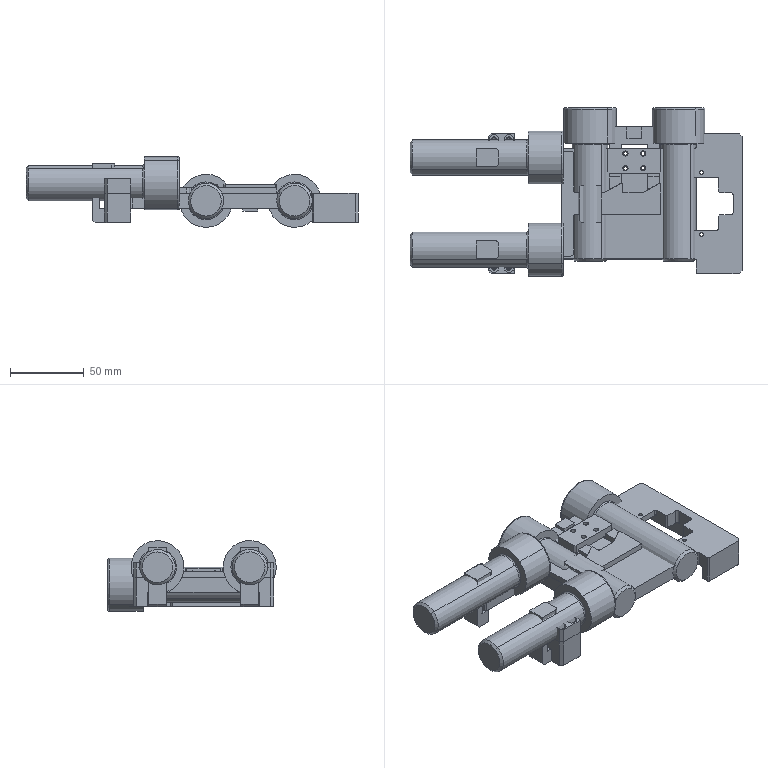Assembly | SolidWorks | mm | 19 component files | 19 solids | 652 faces | box 225 x 114.25 x 48 mm | volume 368375 mm3 | plane 378 | cylinder 216 | cone 34 | torus 16 | spline 8 | commonest cylinder face diameters 5.2 x36 2 x33 2.5 x28 8 x20 4.5 x16 4 x16 3.5 x12 3.3 x8
Bill of materials:
Baffle | 2 |  | Flat annular disc: a thin ring with a concentric through-bore, resembling a plain flat washer.
ClampB | 1 |  | Rectangular block with a stepped top. Two counterbored vertical through-holes sit on the top face, a large horizontal through-bore runs through one side face, and two corners are chamfered in plan.
ClampC | 1 |  | Flat rectangular plate with four through-holes in a rectangular pattern and four chamfered corners.
ConnectingRod | 1 |  | Thin flat profiled plate. A central bar ends in a C-shaped frame on one side, and the other end is a stepped tab with angled shoulders. Small upright posts stand at the four corners of the C-shape.
Jig | 1 |  | Large flat base plate, roughly H/U-shaped in plan, with thicker raised pads at the ends. It has many small and medium through-holes, a stepped rectangular cutout, and narrow slots or rails on the top face.
MirrorClampB1 | 1 |  | Rectangular block with a raised step running along the top. The lower step has two counterbored vertical through-holes, a large horizontal through-bore passes through the taller portion, and two corners are chamfered in plan.
MovingBlock | 2 |  | Bracket-like body: an upright with a rounded top cap, and a horizontal arm projecting sideways that ends in a short upturned tab with a small hole. A small block sits at the base.
PressurePlateA | 1 |  | Rectangular block with two counterbored-looking vertical holes and a wide rectangular channel cut through the underside, giving a bridge or inverted-U cross-section. All plan corners are chamfered.
SideMovingBlock | 1 |  | Complex machined bracket with a long main bar and two parallel legs (a Pi/comb shape in plan). It has multiple through-holes, including a larger central bore, plus end blocks with stepped faces and small raised pads.
socket head cap screw_iso | 4 |  | Cylindrical headed fastener-like part: a plain cylindrical shank with a chamfered tip and a larger cylindrical head with a hexagonal socket recess. It resembles a socket-head cap screw.
VUM5-30 | 2 |  | Open helical coil of round-section wire, about four turns at constant diameter and roughly uniform pitch, with plain cut ends; shape matches a helical coil spring.
VUM5-30 | 2 |  | Open helical coil of round-section wire, about four turns at constant diameter and uniform pitch, with plain flat cut ends; shape matches a helical coil spring, with wire that looks slightly thinner relative to the coil diameter than part-0.
Mates:
1. coincident | Jig-1 face at (-86, 27, 7) dir (0, 0, 1) | MovingBlock-1 face at (-64, 35.5, 7) dir (0, 0, -1)
2. coincident | Jig-1 face at (-86, 27, 7) dir (0, 1, 0) | MovingBlock-1 face at (-64, 27, 10) dir (0, -1, 0)
3. distance | MovingBlock-1 face at (-64, 35.5, 7) dir (1, 0, 0) | Jig-1 face at (-56, 35.5, 7) dir (-1, 0, 0)
4. coincident | Jig-1 face at (-86, 47.5, 10) dir (0, 0, 1) | ClampB-1 face at (-86, 25, 10) dir (0, 0, -1)
5. coincident | Jig-1 face at (-86, 25, 10) dir (0, -1, 0) | ClampB-1 face at (-86, 25, 20) dir (0, -1, 0)
6. coincident | Jig-1 face at (-86, -47.5, 10) dir (-1, 0, 0) | ClampB-1 face at (-86, 47.5, 10) dir (-1, 0, 0)
7. coincident | Jig-1 face at (-86, -27, 7) dir (0, 0, 1) | MovingBlock-2 face at (-64, -27, 7) dir (0, 0, -1)
8. coincident | Jig-1 face at (-86, -35.5, 7) dir (0, 1, 0) | MovingBlock-2 face at (-64, -35.5, 10) dir (0, -1, 0)
9. coincident | Jig-1 face at (-86, 47.5, 10) dir (0, 0, 1) | ConnectingRod-1 face at (-64, 35.5, 10) dir (0, 0, -1)
10. coincident | Jig-1 face at (22, 2.5, 5) dir (0, 0, 1) | SideMovingBlock-1 face at (-22, 40.098, 5) dir (0, 0, -1)
11. coincident | Jig-1 face at (-4, 37.5, 5) dir (1, 0, 0) | SideMovingBlock-1 face at (-4, 10.098, 5) dir (-1, 0, 0)
12. coincident | PressurePlateA-1 face at (-24, 12.5, 10) dir (0, 0, -1) | Jig-1 face at (-86, 47.5, 10) dir (0, 0, 1)
13. distance | PressurePlateA-1 face at (-24, -12.5, 10) dir (-1, 0, 0) | Jig-1 face at (-36, 25, 10) dir (-1, 0, 0)
14. distance | socket head cap screw_iso-4 face at (-17, 65, 5) dir (0, 1, 0) | Jig-1 face at (55, 37.5, 10) dir (0, 1, 0)
15. coincident | Jig-1 face at (-86, 47.5, 10) dir (0, 0, 1) | ClampC-1 face at (-5, 37.5, 10) dir (0, 0, -1)
16. coincident | Jig-1 face at (55, 37.5, 10) dir (0, 1, 0) | ClampC-1 face at (31, 37.5, 16) dir (0, 1, 0)
17. concentric | socket head cap screw_iso-3 face at (-3.25, 31.25, 17) dir (1, 0, 0) r 12 | MovingBlock-1 face at (-64, 31.25, 17) dir (1, 0, 0) r 1.25
18. coincident | MovingBlock-1 face at (-67, 27, 20) dir (-1, 0, 0) | VUM5-30-1 face at (-67, 23.7, 17.885) dir (1, 0, 0)
19. coincident | MovingBlock-1 face at (-94, 25.25, -10) dir (-1, 0, 0) | MovingBlock-2 face at (-94, -37.25, -10) dir (-1, 0, 0)
20. distance | socket head cap screw_iso-3 face at (-59, 44.866, 28.773) dir (-1, 0, 0) | MovingBlock-1 face at (-64, 35.5, 7) dir (1, 0, 0)
21. coincident | MovingBlock-1 face at (-64, 35.5, 7) dir (1, 0, 0) | ConnectingRod-1 face at (-64, -35.5, 14) dir (-1, 0, 0)
22. coincident | MovingBlock-1 face at (-64, 35.5, 10) dir (0, 1, 0) | ConnectingRod-1 face at (31, 35.5, 14) dir (0, 1, 0)
23. concentric | ClampB-1 face at (-83, 31, 17) dir (1, 0, 0) r 4 | VUM5-30-1 face at (-66.25, 31, 17) dir (-1, 0, 0) r 2.6
24. coincident | socket head cap screw_iso-3 face at (-35, 31.25, 17) dir (1, 0, 0) | socket head cap screw_iso-2 face at (-35, -31.25, 17) dir (1, 0, 0)
25. concentric | MovingBlock-2 face at (-64, -31.25, 17) dir (1, 0, 0) r 1.25 | socket head cap screw_iso-2 face at (-3.25, -31.25, 17) dir (1, 0, 0) r 12
26. coincident | MovingBlock-2 face at (-67, -35.5, 20) dir (-1, 0, 0) | VUM5-30-2 face at (-67, -23.647, 16.886) dir (1, 0, 0)
27. coincident | ConnectingRod-1 face at (31, 7.5, 9) dir (0, 1, 0) | PressurePlateA-1 face at (-24, 7.5, 14) dir (0, -1, 0)
28. coincident | ConnectingRod-1 face at (29.392, 13.5, 10) dir (-0.5, 0.866, 0) | SideMovingBlock-1 face at (30, 13.851, 10) dir (0.5, -0.866, 0)
29. coincident | SideMovingBlock-1 face at (-17, 42.098, 5) dir (0, 1, 0) | VUM5-30-3 face at (-9.649, 42.098, 4.798) dir (0, -1, 0)
30. concentric | SideMovingBlock-1 face at (-17, 42.098, 5) dir (0, 1, 0) r 4 | VUM5-30-3 face at (-17, 62.25, 5) dir (0, -1, 0) r 2.6
31. concentric | SideMovingBlock-1 face at (-17, 42.098, 5) dir (0, 1, 0) r 4 | socket head cap screw_iso-4 face at (-17, 96.75, 5) dir (0, 1, 0) r 12
32. concentric | SideMovingBlock-1 face at (43, 42.098, 5) dir (0, 1, 0) r 4 | socket head cap screw_iso-5 face at (43, 96.75, 5) dir (0, 1, 0) r 12
33. coincident | SideMovingBlock-1 face at (43, 42.098, 5) dir (0, 1, 0) | VUM5-30-4 face at (50.351, 42.098, 4.798) dir (0, -1, 0)
34. concentric | SideMovingBlock-1 face at (43, 42.098, 5) dir (0, 1, 0) r 4 | VUM5-30-4 face at (43, 62.25, 5) dir (0, -1, 0) r 2.6
35. distance | ClampC-1 face at (31, 20.5, 16) dir (1, 0, 0) | SideMovingBlock-1 face at (30, 10.098, 5) dir (1, 0, 0)
36. coincident | socket head cap screw_iso-4 face at (-17, 65, 5) dir (0, 1, 0) | socket head cap screw_iso-5 face at (43, 65, 5) dir (0, 1, 0)
37. coincident | socket head cap screw_iso-4 face at (-30.616, 41, 16.773) dir (0, -1, 0) | Baffle-1 face at (-17, 41, 5) dir (0, 1, 0)
38. concentric | socket head cap screw_iso-4 face at (-17, 96.75, 5) dir (0, 1, 0) r 12 | Baffle-1 face at (-17, 39.5, 5) dir (0, 1, 0) r 5
39. concentric | socket head cap screw_iso-5 face at (43, 96.75, 5) dir (0, 1, 0) r 12 | Baffle-2 face at (43, 39.5, 5) dir (0, 1, 0) r 2.25
40. coincident | socket head cap screw_iso-5 face at (29.384, 41, 16.773) dir (0, -1, 0) | Baffle-2 face at (43, 41, 5) dir (0, 1, 0)
41. concentric | Jig-1 face at (-82, -43.5, 10) dir (0, 0, 1) r 1.25 | MirrorClampB1-1 face at (-82, -43.5, 20) dir (0, 0, 1) r 1.7
42. concentric | Jig-1 face at (-72, -43.5, 10) dir (0, 0, 1) r 1.25 | MirrorClampB1-1 face at (-72, -43.5, 20) dir (0, 0, 1) r 1.7
43. coincident | Jig-1 face at (-86, 47.5, 10) dir (0, 0, 1) | MirrorClampB1-1 face at (-86, -25, 10) dir (0, 0, -1)
44. concentric | MirrorClampB1-1 face at (-83, -31, 17) dir (1, 0, 0) r 4 | VUM5-30-2 face at (-66.25, -31, 17) dir (-1, 0, 0) r 2.6